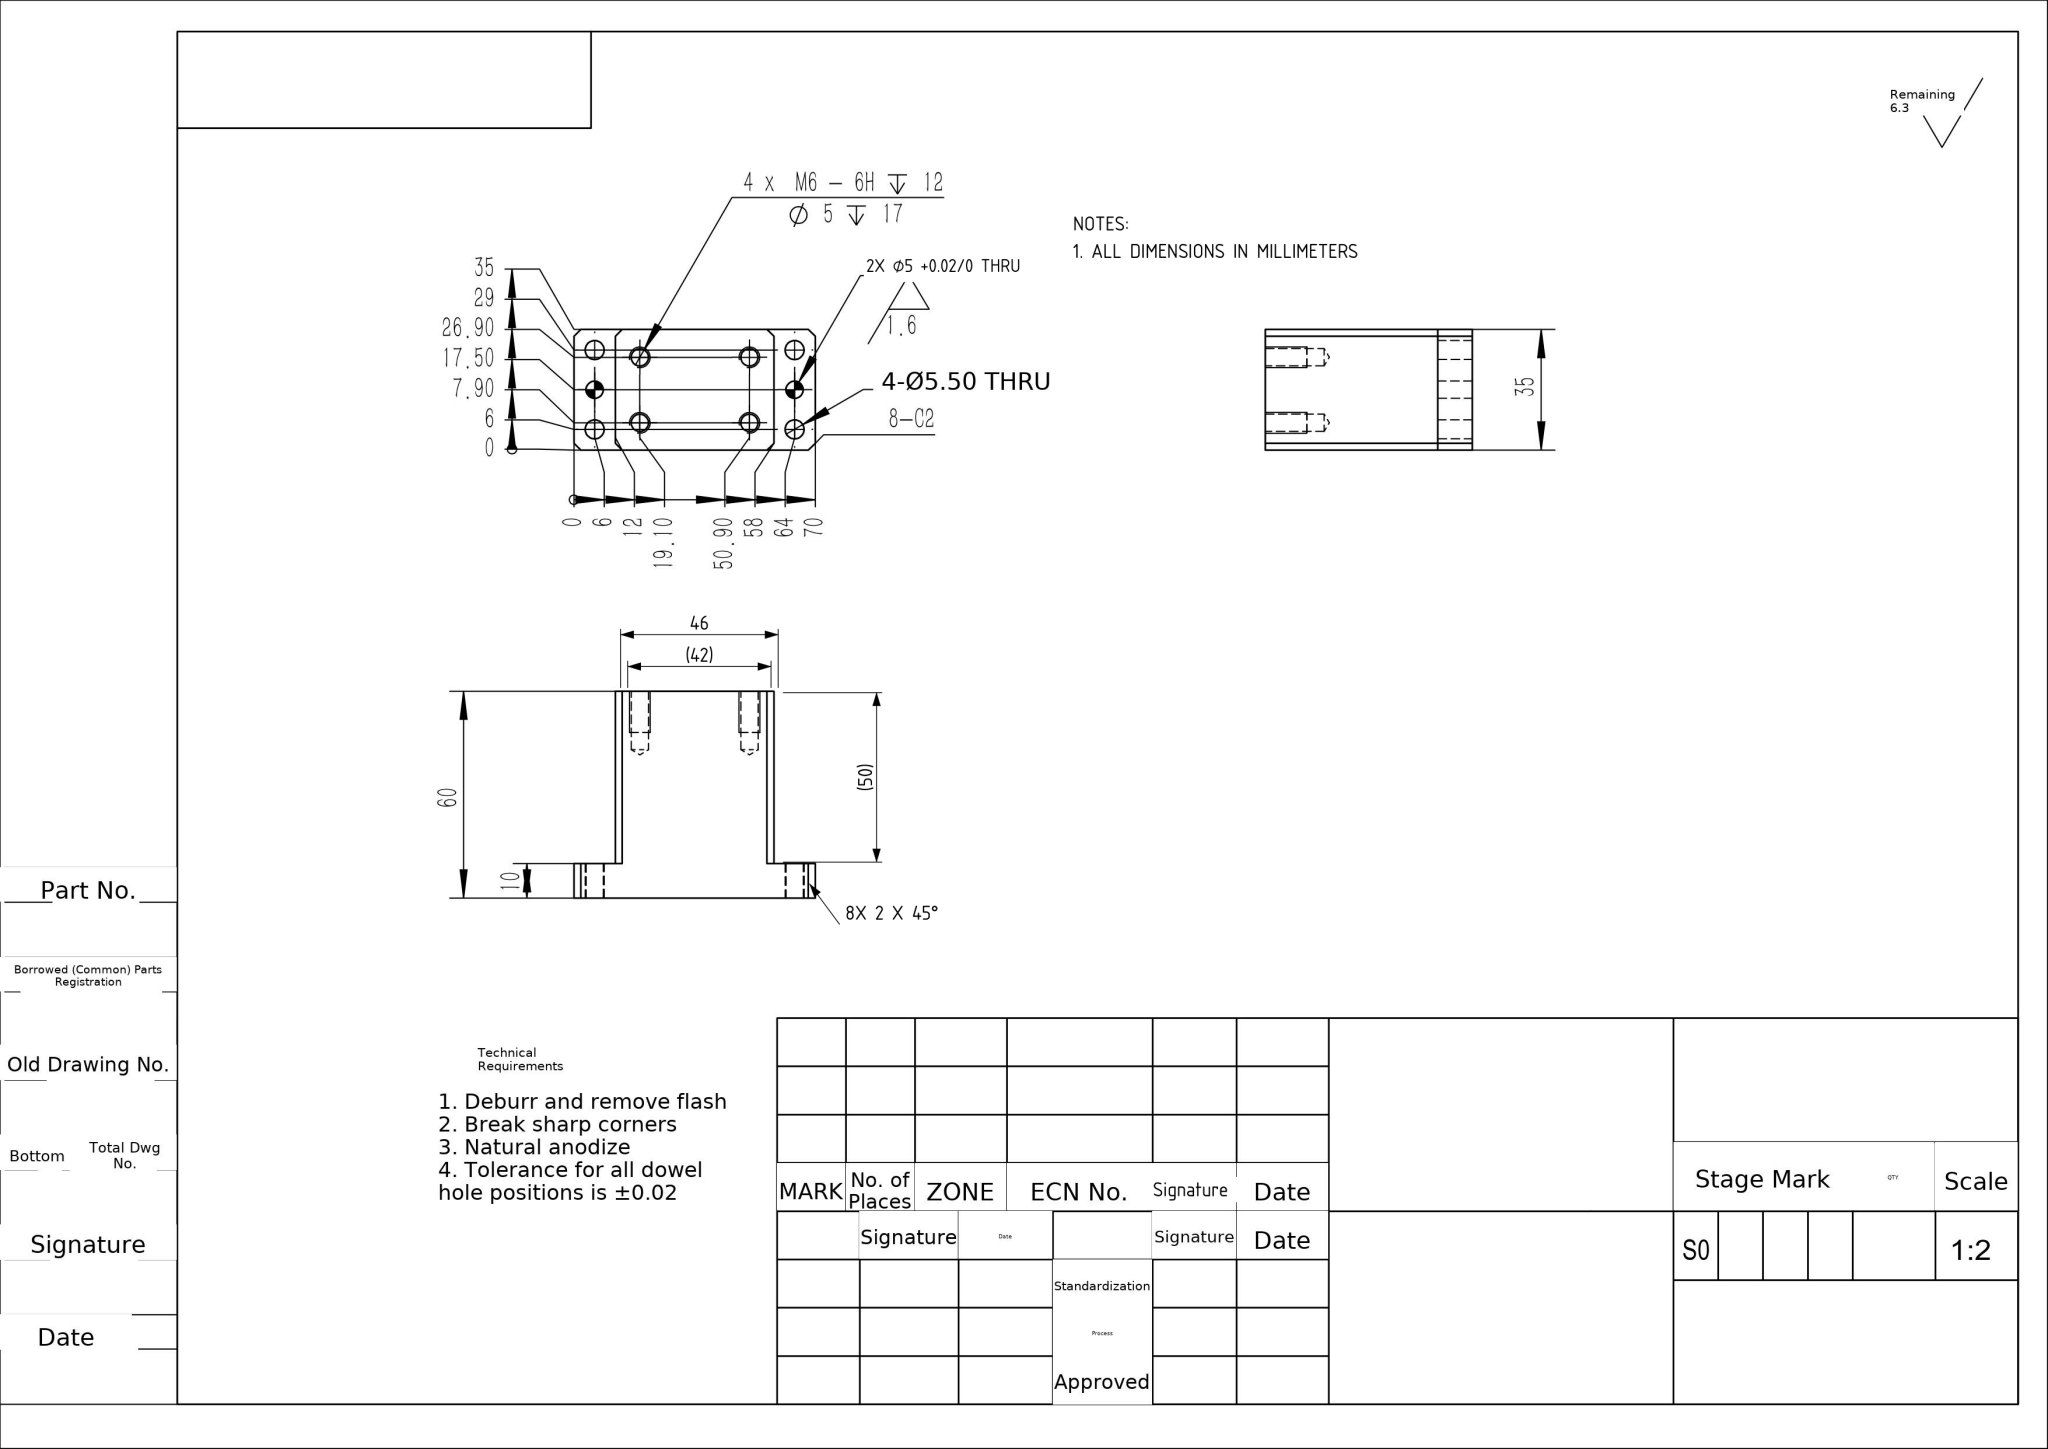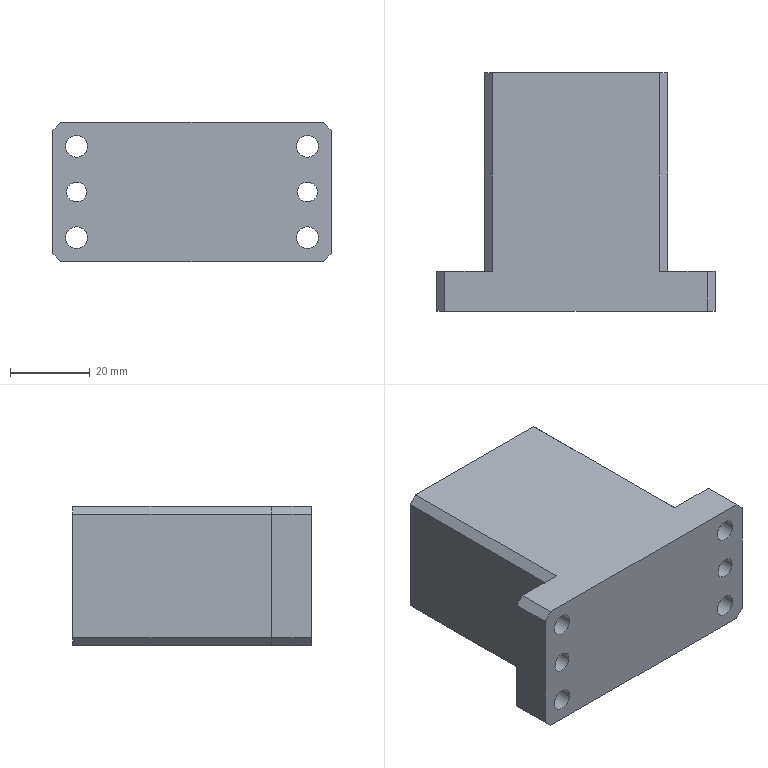Part | NX | mm | 1 solid | 36 faces | box 70 x 60 x 35 mm | volume 101912 mm3 | plane 18 | cylinder 10 | cone 8 | commonest cylinder face diameters 5 x6 5.5 x4